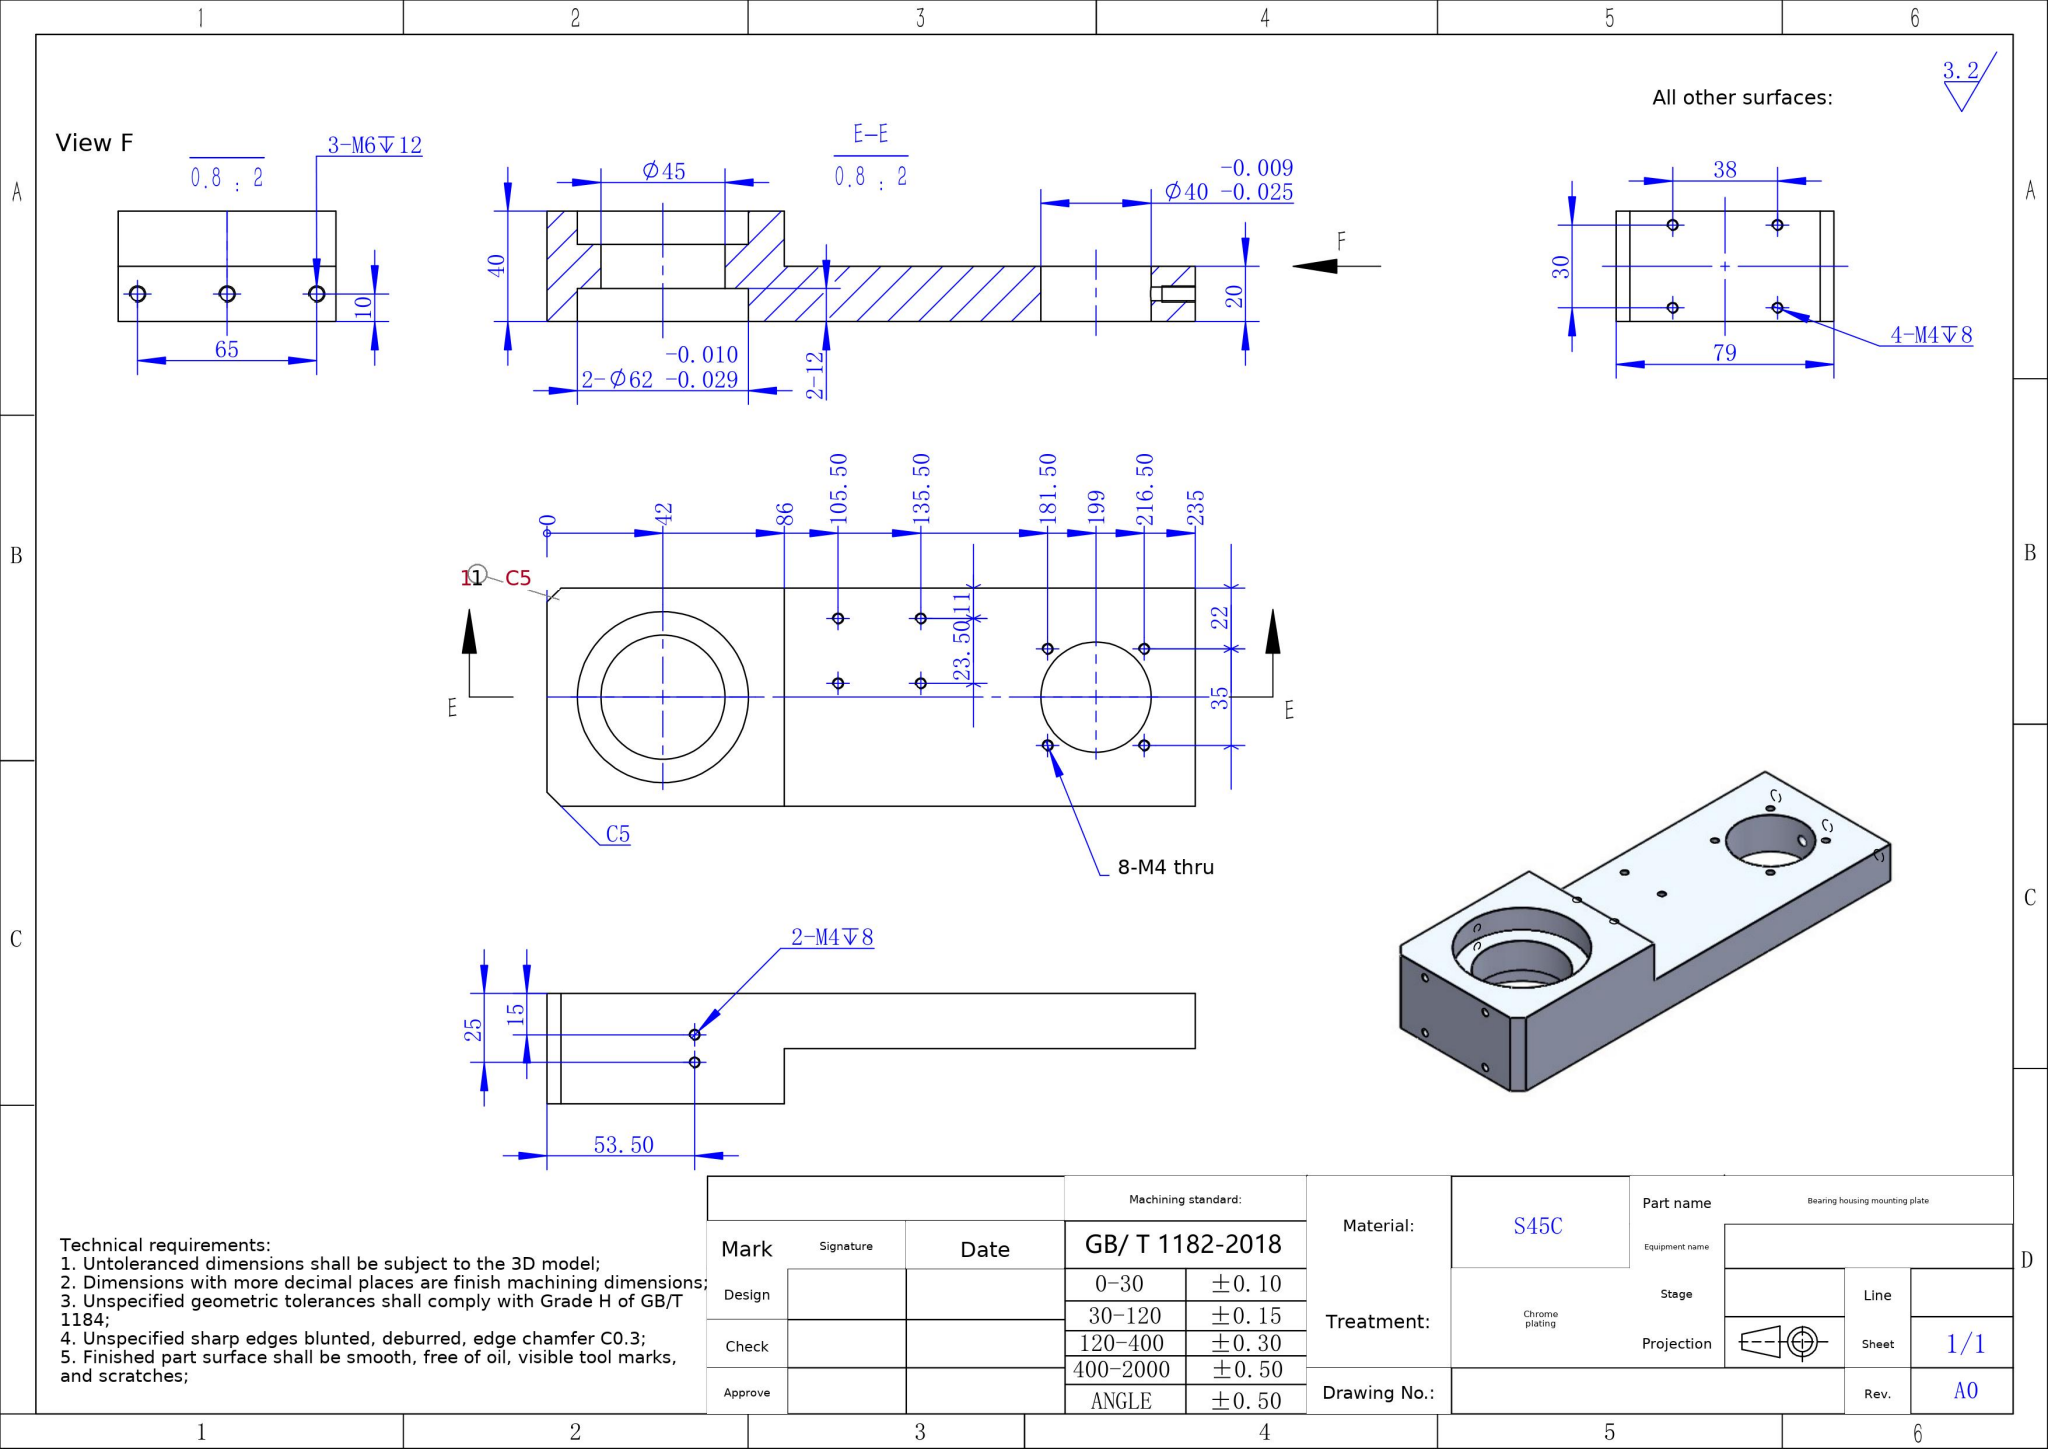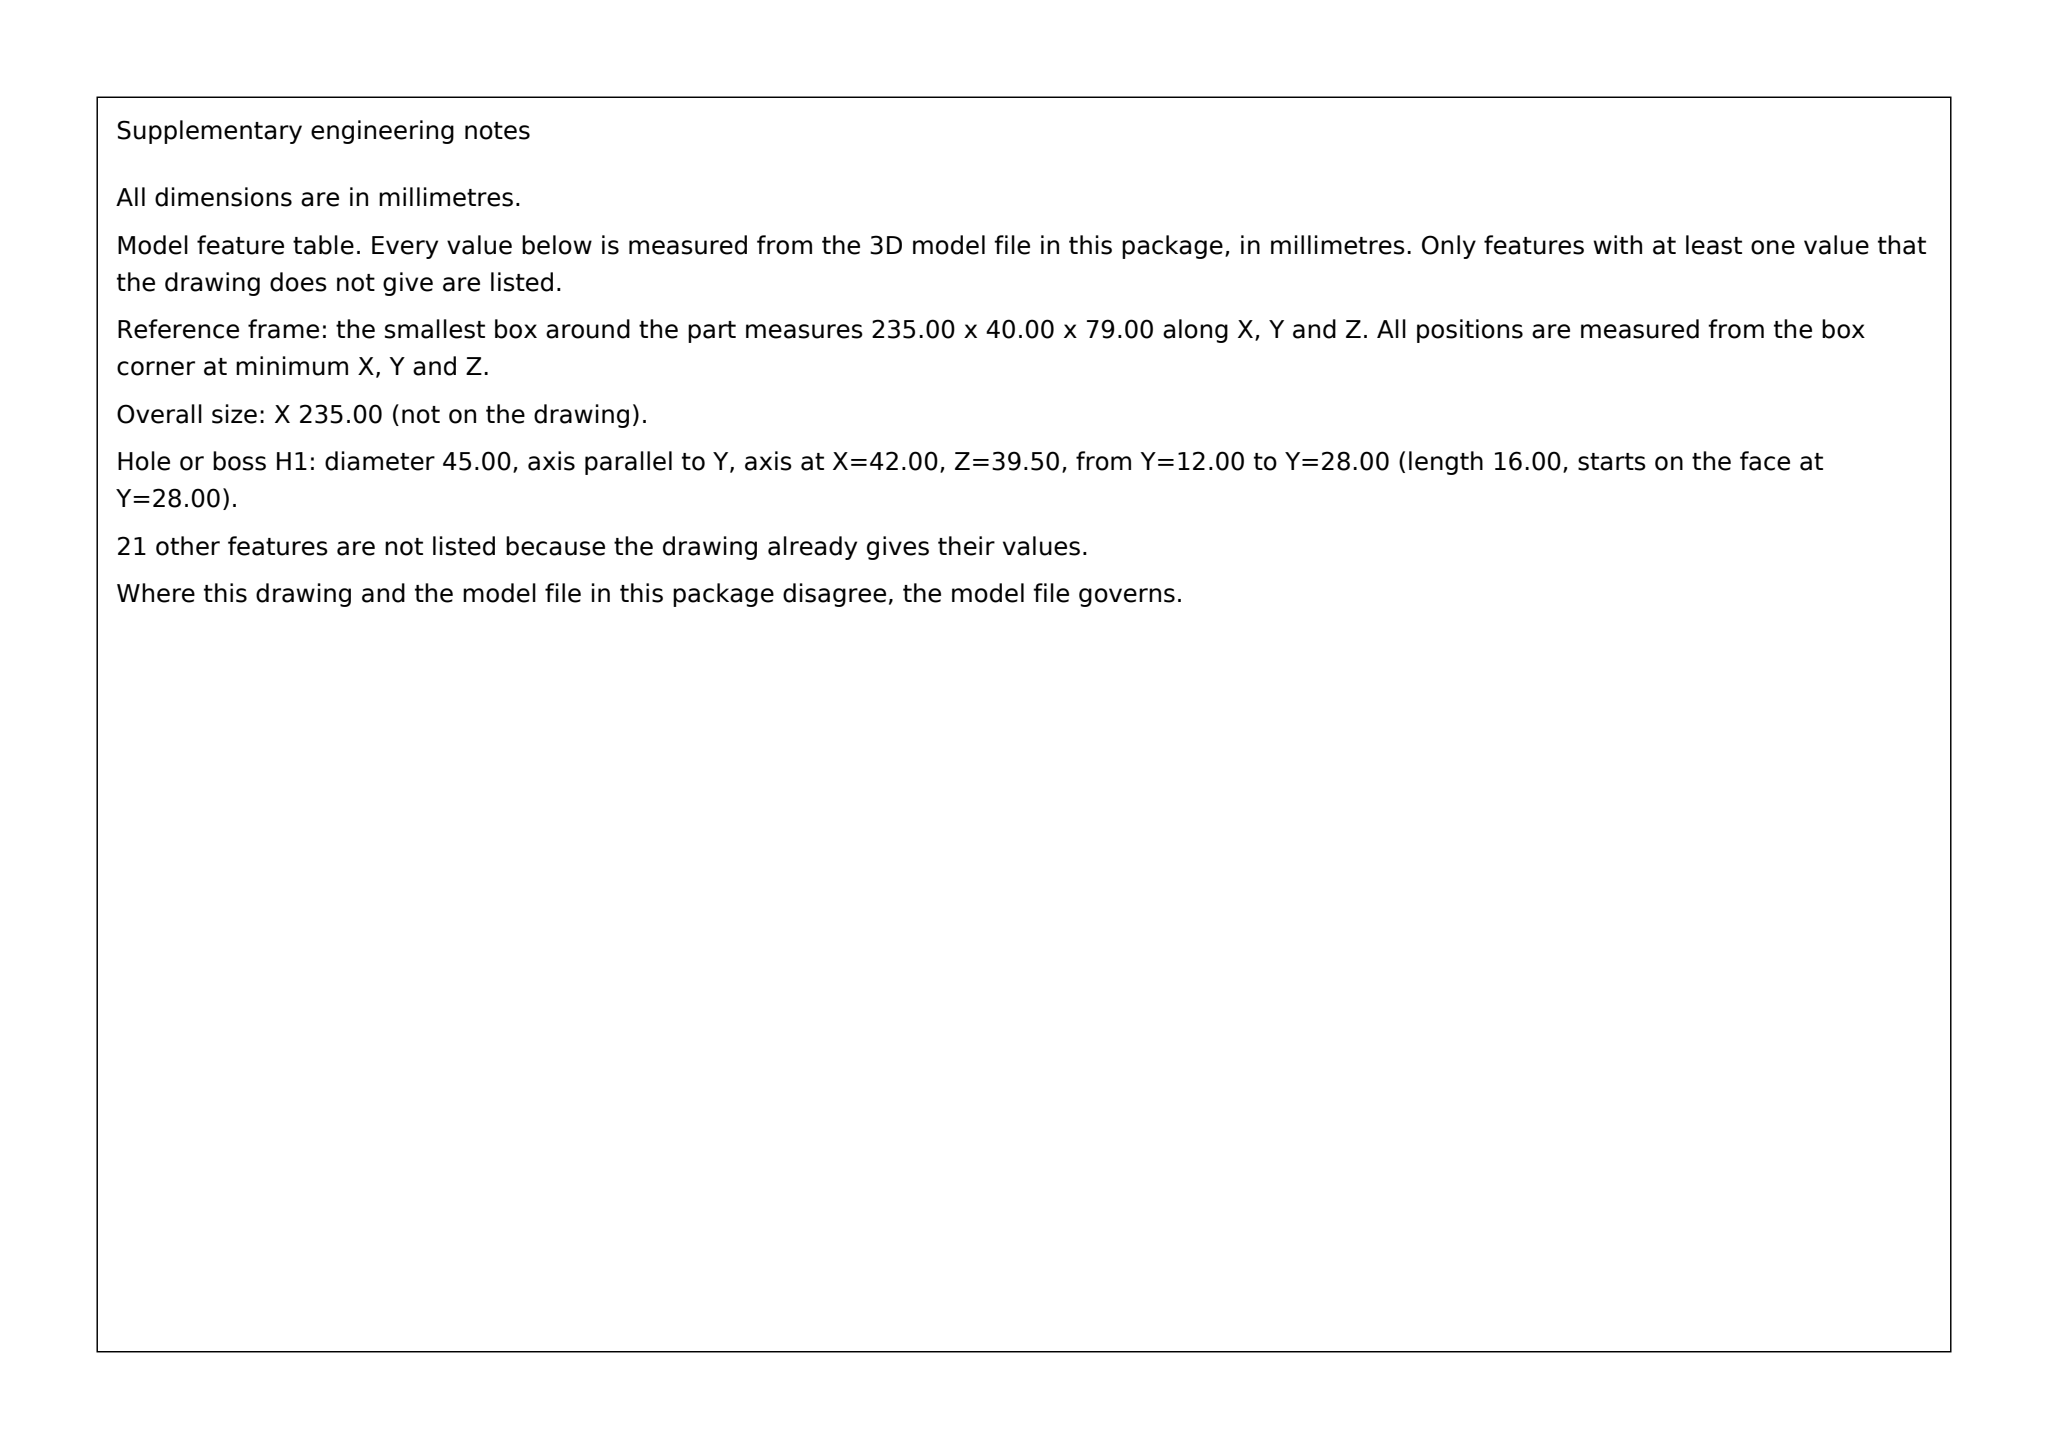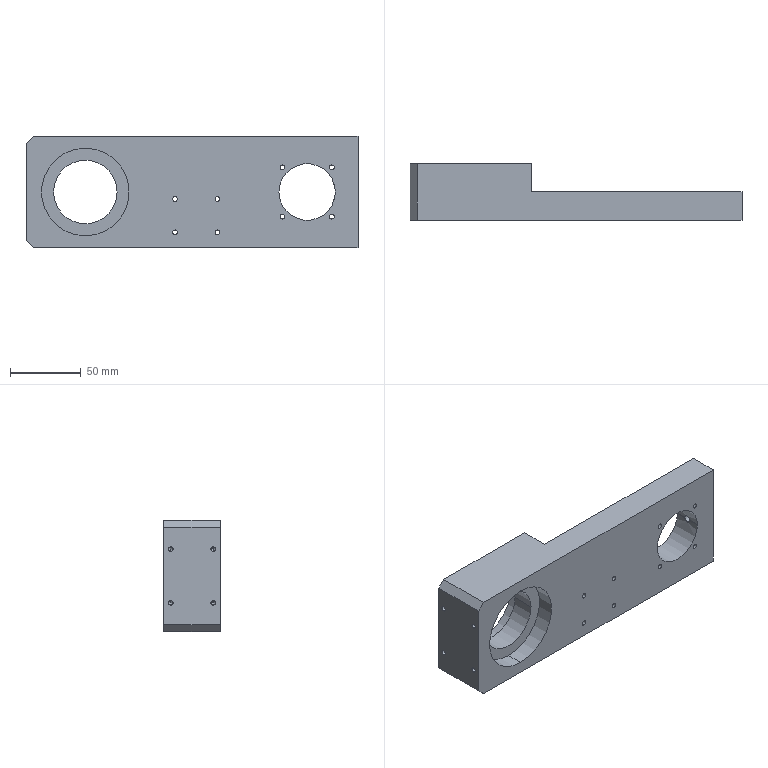Part | SolidWorks | mm | material S45C | 1 solid | 70 faces | box 235 x 40 x 79 mm | volume 380165 mm3 | cylinder 42 | cone 16 | plane 12 | commonest cylinder face diameters 3.3 x28 5 x6 62 x4 40 x2 45 x2